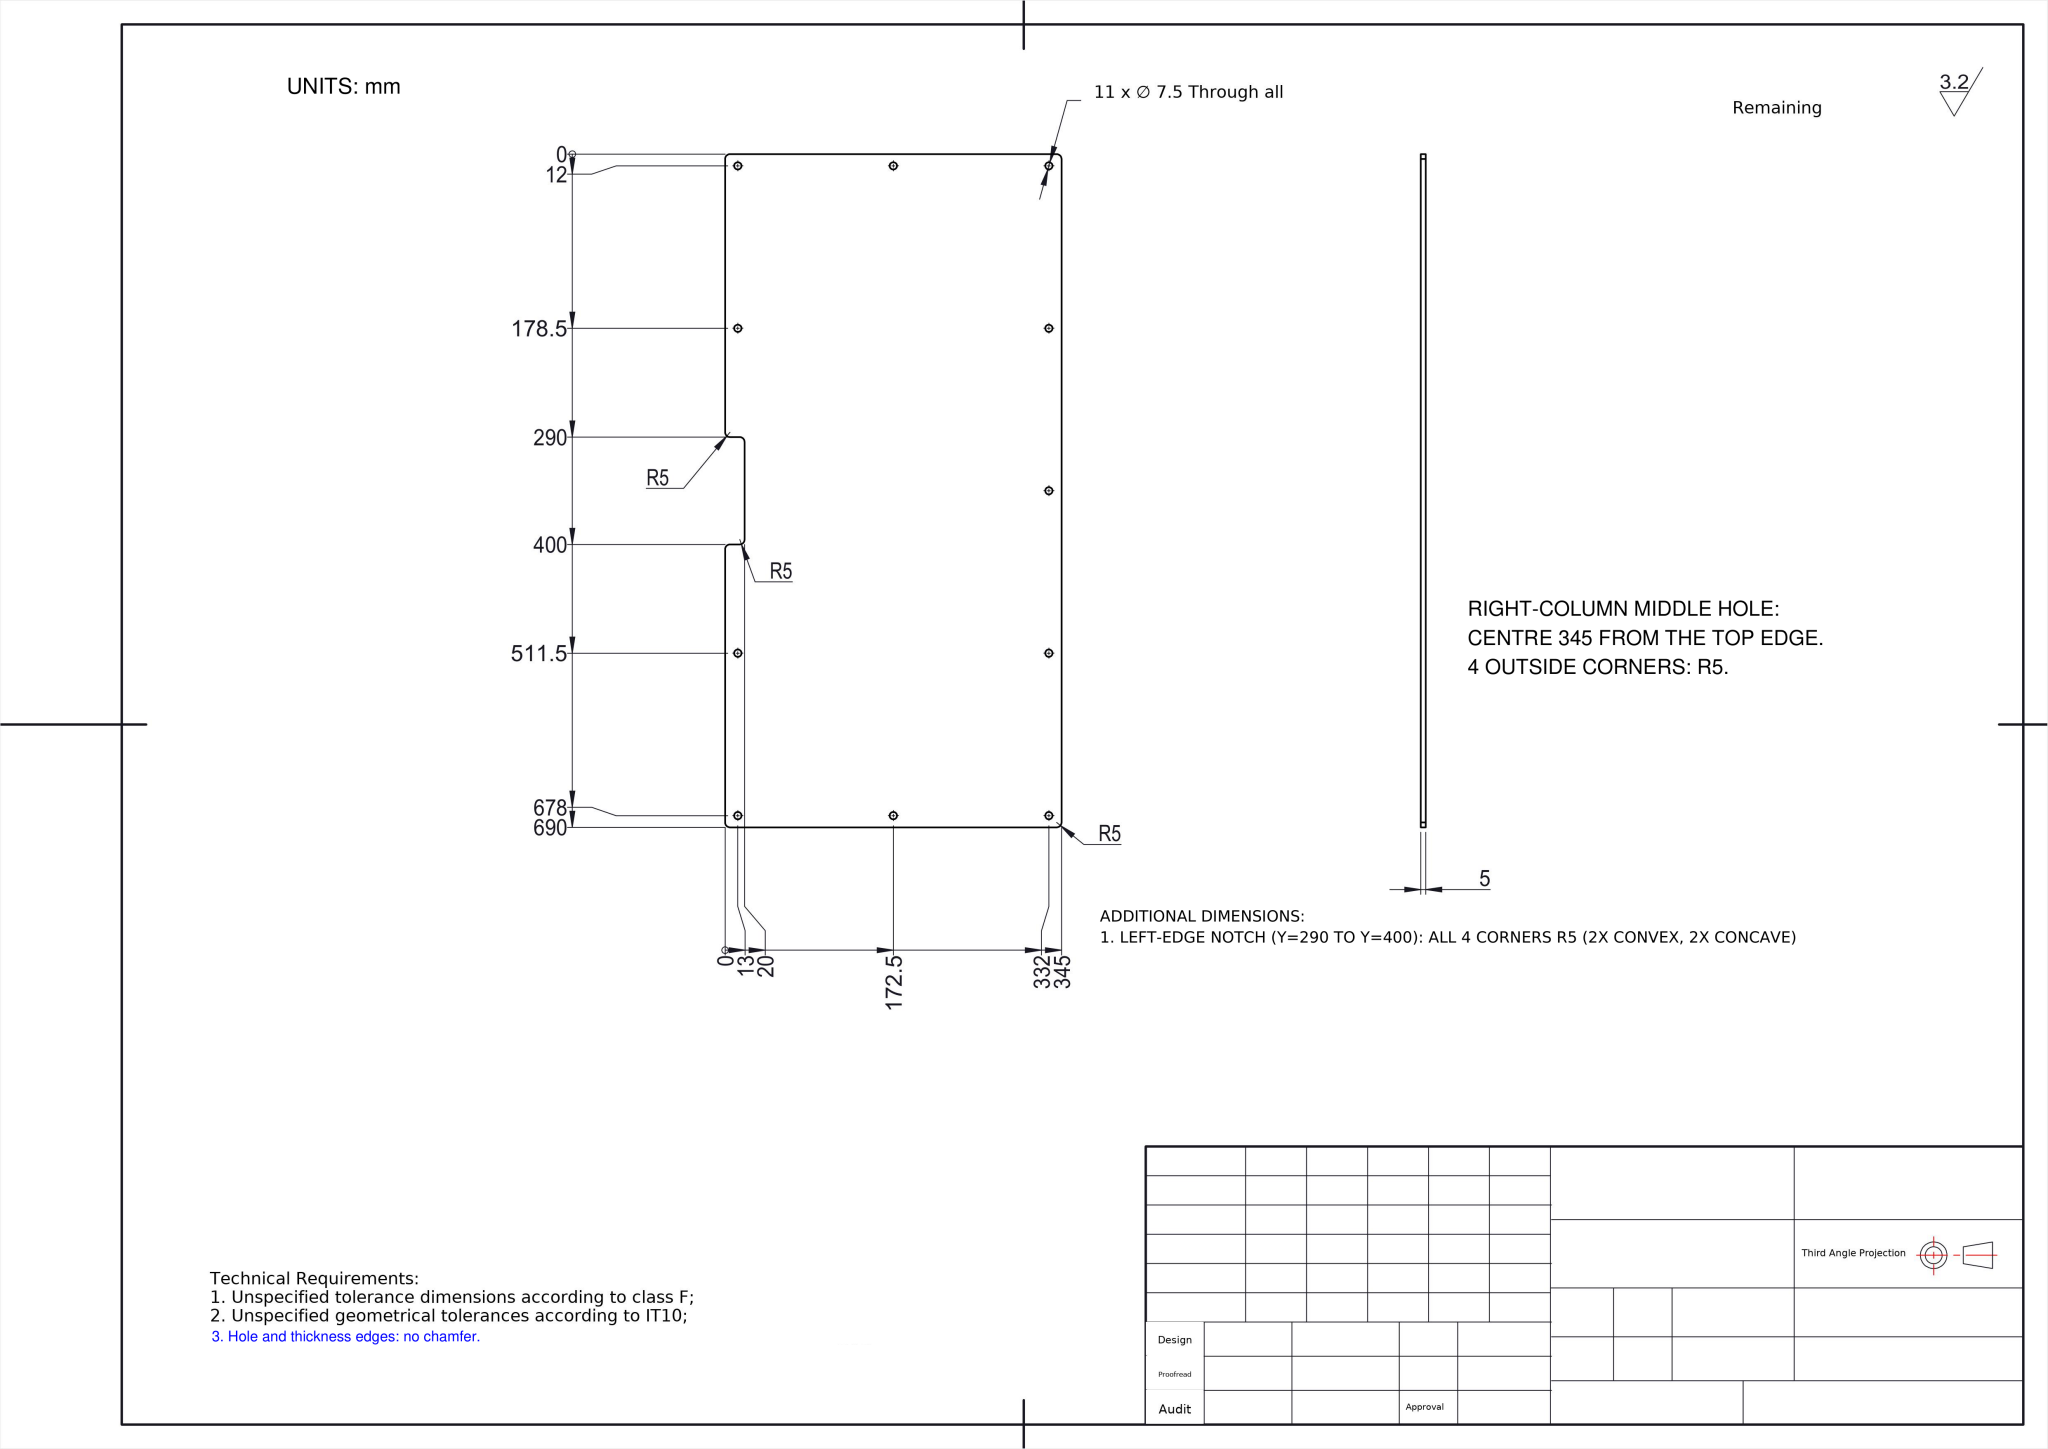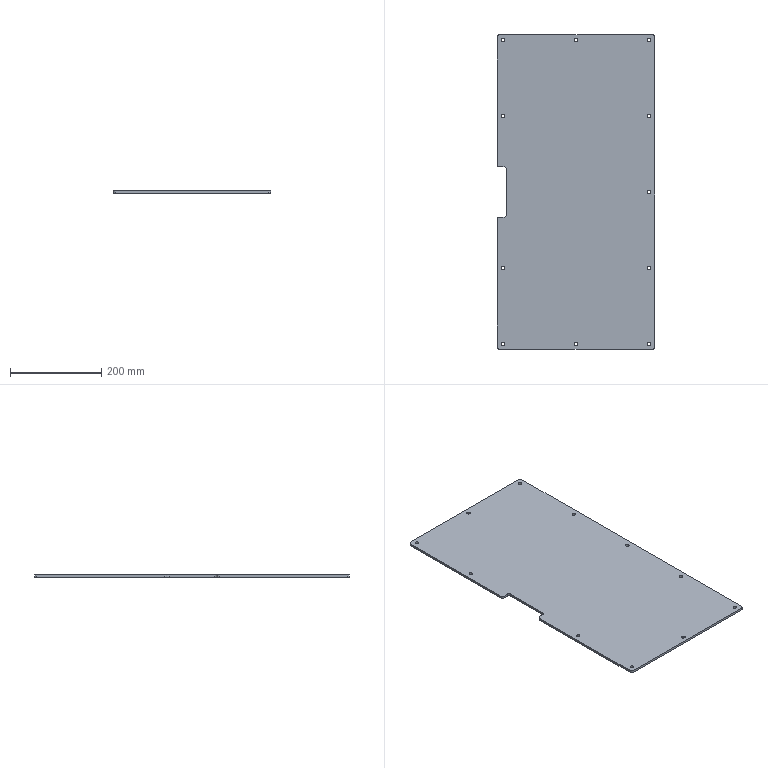Part | NX | mm | 1 solid | 40 faces | box 345 x 690 x 5 mm | volume 1176713 mm3 | cylinder 30 | plane 10 | commonest cylinder face diameters 7.5 x22 10 x8